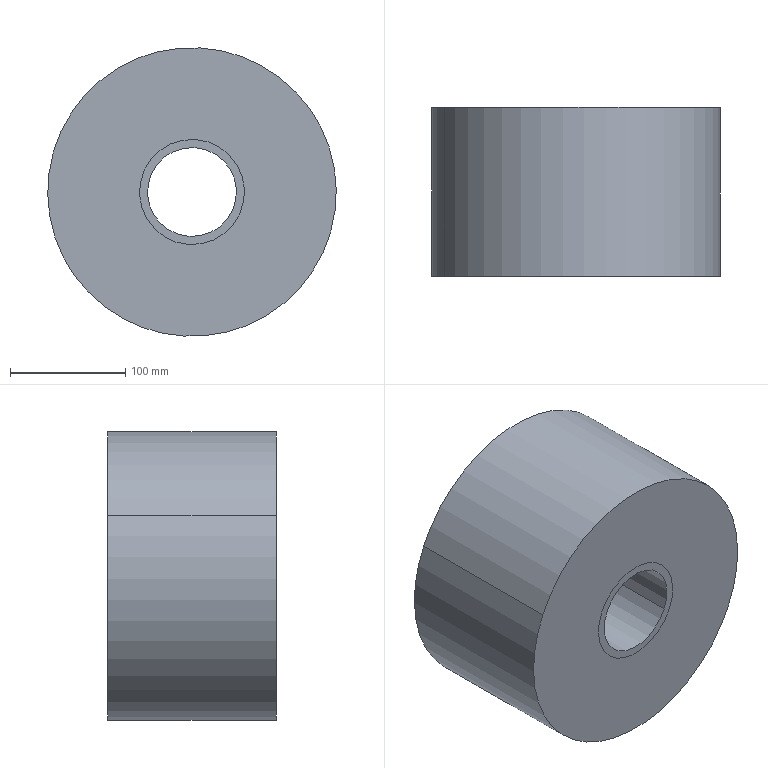Component | SolidWorks | ProtectiveFilm-4 | 2 solids | 12 faces | box 250 x 146 x 250 mm | volume 6486891 mm3 | cylinder 8 | plane 4 | commonest cylinder face diameters 91 x4 250 x2 77 x2
build123d program:
from build123d import *

# Parameters (mm, degrees)
SKETCH1_R           = 45.5
SKETCH1_R_2         = 38.5
BOSS_EXTRUDE1_DEPTH = 146
SKETCH2_R           = 125
SKETCH2_R_2         = 45.5
BOSS_EXTRUDE2_DEPTH = 146


with BuildPart() as part:
    # Sketch1 → Boss-Extrude1 (new body)
    with BuildSketch(Plane.XY):
        Circle(SKETCH1_R)
        Circle(SKETCH1_R_2, mode=Mode.SUBTRACT)
    extrude(amount=BOSS_EXTRUDE1_DEPTH)


with BuildPart() as body_2:
    # Sketch2 → Boss-Extrude2 (new body)
    with BuildSketch(Plane.XY):
        Circle(SKETCH2_R)
        Circle(SKETCH2_R_2, mode=Mode.SUBTRACT)
    extrude(amount=BOSS_EXTRUDE2_DEPTH)


solid = Compound([part.part, body_2.part])

# Placed as in the assembly
solid = solid.moved(Location((50, 183.5, 340), (90, 0, 0)))
STEP:
#1=COLOUR_RGB('',0.7922,0.8196,0.9333);
#2=FILL_AREA_STYLE_COLOUR('',#1);
#3=FILL_AREA_STYLE('',(#2));
#4=SURFACE_STYLE_FILL_AREA(#3);
#5=SURFACE_SIDE_STYLE('',(#4));
#6=SURFACE_STYLE_USAGE(.BOTH.,#5);
#7=PRESENTATION_STYLE_ASSIGNMENT((#6));
#8=CARTESIAN_POINT('',(0.3406,7.224,14.133));
#9=VERTEX_POINT('',#8);
#10=CARTESIAN_POINT('',(3.596,7.224,12.638));
#11=VERTEX_POINT('',#10);
#12=CARTESIAN_POINT('',(1.969,7.224,13.386));
#13=DIRECTION('',(0.,1.,0.));
#14=DIRECTION('',(0.9087,0.,-0.4174));
#15=AXIS2_PLACEMENT_3D('',#12,#13,#14);
#16=CIRCLE('',#15,1.791);
#17=EDGE_CURVE('',#9,#11,#16,.T.);
#18=ORIENTED_EDGE('',*,*,#17,.T.);
#19=CARTESIAN_POINT('',(3.596,1.476,12.638));
#20=VERTEX_POINT('',#19);
#21=CARTESIAN_POINT('',(3.596,7.224,12.638));
#22=DIRECTION('',(0.,-1.,0.));
#23=VECTOR('',#22,39.37);
#24=LINE('',#21,#23);
#25=EDGE_CURVE('',#11,#20,#24,.T.);
#26=ORIENTED_EDGE('',*,*,#25,.T.);
#27=CARTESIAN_POINT('',(0.3406,1.476,14.133));
#28=VERTEX_POINT('',#27);
#29=CARTESIAN_POINT('',(1.969,1.476,13.386));
#30=DIRECTION('',(0.,1.,0.));
#31=DIRECTION('',(0.9087,0.,-0.4174));
#32=AXIS2_PLACEMENT_3D('',#29,#30,#31);
#33=CIRCLE('',#32,1.791);
#34=EDGE_CURVE('',#28,#20,#33,.T.);
#35=ORIENTED_EDGE('',*,*,#34,.F.);
#36=CARTESIAN_POINT('',(0.3406,7.224,14.133));
#37=DIRECTION('',(0.,-1.,0.));
#38=VECTOR('',#37,39.37);
#39=LINE('',#36,#38);
#40=EDGE_CURVE('',#9,#28,#39,.T.);
#41=ORIENTED_EDGE('',*,*,#40,.F.);
#42=EDGE_LOOP('',(#18,#26,#35,#41));
#43=FACE_OUTER_BOUND('',#42,.T.);
#44=CARTESIAN_POINT('',(1.969,7.224,13.386));
#45=DIRECTION('',(0.,-1.,0.));
#46=DIRECTION('',(-0.9087,0.,0.4174));
#47=AXIS2_PLACEMENT_3D('',#44,#45,#46);
#48=CYLINDRICAL_SURFACE('',#47,1.791);
#49=ADVANCED_FACE('',(#43),#48,.F.);
#50=CARTESIAN_POINT('',(6.441,7.224,11.332));
#51=VERTEX_POINT('',#50);
#52=CARTESIAN_POINT('',(-2.504,7.224,15.44));
#53=VERTEX_POINT('',#52);
#54=CARTESIAN_POINT('',(1.969,7.224,13.386));
#55=DIRECTION('',(0.,1.,0.));
#56=DIRECTION('',(0.9087,0.,-0.4174));
#57=AXIS2_PLACEMENT_3D('',#54,#55,#56);
#58=CIRCLE('',#57,4.921);
#59=EDGE_CURVE('',#51,#53,#58,.T.);
#60=ORIENTED_EDGE('',*,*,#59,.F.);
#61=CARTESIAN_POINT('',(6.441,1.476,11.332));
#62=VERTEX_POINT('',#61);
#63=CARTESIAN_POINT('',(6.441,7.224,11.332));
#64=DIRECTION('',(0.,-1.,0.));
#65=VECTOR('',#64,39.37);
#66=LINE('',#63,#65);
#67=EDGE_CURVE('',#51,#62,#66,.T.);
#68=ORIENTED_EDGE('',*,*,#67,.T.);
#69=CARTESIAN_POINT('',(-2.504,1.476,15.44));
#70=VERTEX_POINT('',#69);
#71=CARTESIAN_POINT('',(1.969,1.476,13.386));
#72=DIRECTION('',(0.,1.,0.));
#73=DIRECTION('',(0.9087,0.,-0.4174));
#74=AXIS2_PLACEMENT_3D('',#71,#72,#73);
#75=CIRCLE('',#74,4.921);
#76=EDGE_CURVE('',#62,#70,#75,.T.);
#77=ORIENTED_EDGE('',*,*,#76,.T.);
#78=CARTESIAN_POINT('',(-2.504,7.224,15.44));
#79=DIRECTION('',(0.,-1.,0.));
#80=VECTOR('',#79,39.37);
#81=LINE('',#78,#80);
#82=EDGE_CURVE('',#53,#70,#81,.T.);
#83=ORIENTED_EDGE('',*,*,#82,.F.);
#84=EDGE_LOOP('',(#60,#68,#77,#83));
#85=FACE_OUTER_BOUND('',#84,.T.);
#86=CARTESIAN_POINT('',(1.969,7.224,13.386));
#87=DIRECTION('',(0.,-1.,0.));
#88=DIRECTION('',(-0.9087,0.,0.4174));
#89=AXIS2_PLACEMENT_3D('',#86,#87,#88);
#90=CYLINDRICAL_SURFACE('',#89,4.921);
#91=ADVANCED_FACE('',(#85),#90,.T.);
#92=CARTESIAN_POINT('',(1.969,7.224,13.386));
#93=DIRECTION('',(0.,1.,0.));
#94=DIRECTION('',(0.9087,0.,-0.4174));
#95=AXIS2_PLACEMENT_3D('',#92,#93,#94);
#96=CIRCLE('',#95,4.921);
#97=EDGE_CURVE('',#53,#51,#96,.T.);
#98=ORIENTED_EDGE('',*,*,#97,.T.);
#99=ORIENTED_EDGE('',*,*,#59,.T.);
#100=EDGE_LOOP('',(#98,#99));
#101=FACE_OUTER_BOUND('',#100,.T.);
#102=ORIENTED_EDGE('',*,*,#17,.F.);
#103=CARTESIAN_POINT('',(1.969,7.224,13.386));
#104=DIRECTION('',(0.,1.,0.));
#105=DIRECTION('',(0.9087,0.,-0.4174));
#106=AXIS2_PLACEMENT_3D('',#103,#104,#105);
#107=CIRCLE('',#106,1.791);
#108=EDGE_CURVE('',#11,#9,#107,.T.);
#109=ORIENTED_EDGE('',*,*,#108,.F.);
#110=EDGE_LOOP('',(#102,#109));
#111=FACE_BOUND('',#110,.T.);
#112=CARTESIAN_POINT('',(1.969,7.224,13.386));
#113=DIRECTION('',(0.,1.,0.));
#114=DIRECTION('',(0.9087,0.,-0.4174));
#115=AXIS2_PLACEMENT_3D('',#112,#113,#114);
#116=PLANE('',#115);
#117=ADVANCED_FACE('',(#101,#111),#116,.T.);
#118=CARTESIAN_POINT('',(1.969,1.476,13.386));
#119=DIRECTION('',(0.,1.,0.));
#120=DIRECTION('',(0.9087,0.,-0.4174));
#121=AXIS2_PLACEMENT_3D('',#118,#119,#120);
#122=CIRCLE('',#121,4.921);
#123=EDGE_CURVE('',#70,#62,#122,.T.);
#124=ORIENTED_EDGE('',*,*,#123,.F.);
#125=ORIENTED_EDGE('',*,*,#76,.F.);
#126=EDGE_LOOP('',(#124,#125));
#127=FACE_OUTER_BOUND('',#126,.T.);
#128=ORIENTED_EDGE('',*,*,#34,.T.);
#129=CARTESIAN_POINT('',(1.969,1.476,13.386));
#130=DIRECTION('',(0.,1.,0.));
#131=DIRECTION('',(0.9087,0.,-0.4174));
#132=AXIS2_PLACEMENT_3D('',#129,#130,#131);
#133=CIRCLE('',#132,1.791);
#134=EDGE_CURVE('',#20,#28,#133,.T.);
#135=ORIENTED_EDGE('',*,*,#134,.T.);
#136=EDGE_LOOP('',(#128,#135));
#137=FACE_BOUND('',#136,.T.);
#138=CARTESIAN_POINT('',(1.969,1.476,13.386));
#139=DIRECTION('',(0.,1.,0.));
#140=DIRECTION('',(0.9087,0.,-0.4174));
#141=AXIS2_PLACEMENT_3D('',#138,#139,#140);
#142=PLANE('',#141);
#143=ADVANCED_FACE('',(#127,#137),#142,.F.);
#144=ORIENTED_EDGE('',*,*,#67,.F.);
#145=ORIENTED_EDGE('',*,*,#97,.F.);
#146=ORIENTED_EDGE('',*,*,#82,.T.);
#147=ORIENTED_EDGE('',*,*,#123,.T.);
#148=EDGE_LOOP('',(#144,#145,#146,#147));
#149=FACE_OUTER_BOUND('',#148,.T.);
#150=CARTESIAN_POINT('',(1.969,7.224,13.386));
#151=DIRECTION('',(0.,-1.,0.));
#152=DIRECTION('',(-0.9087,0.,0.4174));
#153=AXIS2_PLACEMENT_3D('',#150,#151,#152);
#154=CYLINDRICAL_SURFACE('',#153,4.921);
#155=ADVANCED_FACE('',(#149),#154,.T.);
#156=ORIENTED_EDGE('',*,*,#25,.F.);
#157=ORIENTED_EDGE('',*,*,#108,.T.);
#158=ORIENTED_EDGE('',*,*,#40,.T.);
#159=ORIENTED_EDGE('',*,*,#134,.F.);
#160=EDGE_LOOP('',(#156,#157,#158,#159));
#161=FACE_OUTER_BOUND('',#160,.T.);
#162=CARTESIAN_POINT('',(1.969,7.224,13.386));
#163=DIRECTION('',(0.,-1.,0.));
#164=DIRECTION('',(-0.9087,0.,0.4174));
#165=AXIS2_PLACEMENT_3D('',#162,#163,#164);
#166=CYLINDRICAL_SURFACE('',#165,1.791);
#167=ADVANCED_FACE('',(#161),#166,.F.);
#168=CLOSED_SHELL('',(#49,#91,#117,#143,#155,#167));
#169=MANIFOLD_SOLID_BREP('',#168);
#170=STYLED_ITEM('',(#7),#169);
#171=(LENGTH_UNIT()NAMED_UNIT(*)SI_UNIT($,.METRE.));
#172=LENGTH_MEASURE_WITH_UNIT(LENGTH_MEASURE(0.0254),#171);
#173=DIMENSIONAL_EXPONENTS(1.,0.,0.,0.,0.,0.,0.);
#174=(CONVERSION_BASED_UNIT('',#172)LENGTH_UNIT()NAMED_UNIT(#173));
#175=UNCERTAINTY_MEASURE_WITH_UNIT(LENGTH_MEASURE(0.00001),#174,'','');
#176=(NAMED_UNIT(*)PLANE_ANGLE_UNIT()SI_UNIT($,.RADIAN.));
#177=(NAMED_UNIT(*)SI_UNIT($,.STERADIAN.)SOLID_ANGLE_UNIT());
#178=(GEOMETRIC_REPRESENTATION_CONTEXT(3)GLOBAL_UNCERTAINTY_ASSIGNED_CONTEXT((#175))GLOBAL_UNIT_ASSIGNED_CONTEXT((#174,#176,#177))REPRESENTATION_CONTEXT('',''));
#179=MECHANICAL_DESIGN_GEOMETRIC_PRESENTATION_REPRESENTATION('',(#170),#178);
#180=PRESENTATION_LAYER_ASSIGNMENT('','',(#170));
#181=CARTESIAN_POINT('',(0.5911,7.224,14.018));
#182=VERTEX_POINT('',#181);
#183=CARTESIAN_POINT('',(3.346,7.224,12.753));
#184=VERTEX_POINT('',#183);
#185=CARTESIAN_POINT('',(1.969,7.224,13.386));
#186=DIRECTION('',(0.,1.,0.));
#187=DIRECTION('',(0.9087,0.,-0.4174));
#188=AXIS2_PLACEMENT_3D('',#185,#186,#187);
#189=CIRCLE('',#188,1.516);
#190=EDGE_CURVE('',#182,#184,#189,.T.);
#191=ORIENTED_EDGE('',*,*,#190,.T.);
#192=CARTESIAN_POINT('',(3.346,1.476,12.753));
#193=VERTEX_POINT('',#192);
#194=CARTESIAN_POINT('',(3.346,7.224,12.753));
#195=DIRECTION('',(0.,-1.,0.));
#196=VECTOR('',#195,39.37);
#197=LINE('',#194,#196);
#198=EDGE_CURVE('',#184,#193,#197,.T.);
#199=ORIENTED_EDGE('',*,*,#198,.T.);
#200=CARTESIAN_POINT('',(0.5911,1.476,14.018));
#201=VERTEX_POINT('',#200);
#202=CARTESIAN_POINT('',(1.969,1.476,13.386));
#203=DIRECTION('',(0.,1.,0.));
#204=DIRECTION('',(0.9087,0.,-0.4174));
#205=AXIS2_PLACEMENT_3D('',#202,#203,#204);
#206=CIRCLE('',#205,1.516);
#207=EDGE_CURVE('',#201,#193,#206,.T.);
#208=ORIENTED_EDGE('',*,*,#207,.F.);
#209=CARTESIAN_POINT('',(0.5911,7.224,14.018));
#210=DIRECTION('',(0.,-1.,0.));
#211=VECTOR('',#210,39.37);
#212=LINE('',#209,#211);
#213=EDGE_CURVE('',#182,#201,#212,.T.);
#214=ORIENTED_EDGE('',*,*,#213,.F.);
#215=EDGE_LOOP('',(#191,#199,#208,#214));
#216=FACE_OUTER_BOUND('',#215,.T.);
#217=CARTESIAN_POINT('',(1.969,7.224,13.386));
#218=DIRECTION('',(0.,-1.,0.));
#219=DIRECTION('',(-0.9087,0.,0.4174));
#220=AXIS2_PLACEMENT_3D('',#217,#218,#219);
#221=CYLINDRICAL_SURFACE('',#220,1.516);
#222=ADVANCED_FACE('',(#216),#221,.F.);
#223=CARTESIAN_POINT('',(3.596,7.224,12.638));
#224=VERTEX_POINT('',#223);
#225=CARTESIAN_POINT('',(0.3406,7.224,14.133));
#226=VERTEX_POINT('',#225);
#227=CARTESIAN_POINT('',(1.969,7.224,13.386));
#228=DIRECTION('',(0.,1.,0.));
#229=DIRECTION('',(0.9087,0.,-0.4174));
#230=AXIS2_PLACEMENT_3D('',#227,#228,#229);
#231=CIRCLE('',#230,1.791);
#232=EDGE_CURVE('',#224,#226,#231,.T.);
#233=ORIENTED_EDGE('',*,*,#232,.F.);
#234=CARTESIAN_POINT('',(3.596,1.476,12.638));
#235=VERTEX_POINT('',#234);
#236=CARTESIAN_POINT('',(3.596,7.224,12.638));
#237=DIRECTION('',(0.,-1.,0.));
#238=VECTOR('',#237,39.37);
#239=LINE('',#236,#238);
#240=EDGE_CURVE('',#224,#235,#239,.T.);
#241=ORIENTED_EDGE('',*,*,#240,.T.);
#242=CARTESIAN_POINT('',(0.3406,1.476,14.133));
#243=VERTEX_POINT('',#242);
#244=CARTESIAN_POINT('',(1.969,1.476,13.386));
#245=DIRECTION('',(0.,1.,0.));
#246=DIRECTION('',(0.9087,0.,-0.4174));
#247=AXIS2_PLACEMENT_3D('',#244,#245,#246);
#248=CIRCLE('',#247,1.791);
#249=EDGE_CURVE('',#235,#243,#248,.T.);
#250=ORIENTED_EDGE('',*,*,#249,.T.);
#251=CARTESIAN_POINT('',(0.3406,7.224,14.133));
#252=DIRECTION('',(0.,-1.,0.));
#253=VECTOR('',#252,39.37);
#254=LINE('',#251,#253);
#255=EDGE_CURVE('',#226,#243,#254,.T.);
#256=ORIENTED_EDGE('',*,*,#255,.F.);
#257=EDGE_LOOP('',(#233,#241,#250,#256));
#258=FACE_OUTER_BOUND('',#257,.T.);
#259=CARTESIAN_POINT('',(1.969,7.224,13.386));
#260=DIRECTION('',(0.,-1.,0.));
#261=DIRECTION('',(-0.9087,0.,0.4174));
#262=AXIS2_PLACEMENT_3D('',#259,#260,#261);
#263=CYLINDRICAL_SURFACE('',#262,1.791);
#264=ADVANCED_FACE('',(#258),#263,.T.);
#265=CARTESIAN_POINT('',(1.969,7.224,13.386));
#266=DIRECTION('',(0.,1.,0.));
#267=DIRECTION('',(0.9087,0.,-0.4174));
#268=AXIS2_PLACEMENT_3D('',#265,#266,#267);
#269=CIRCLE('',#268,1.791);
#270=EDGE_CURVE('',#226,#224,#269,.T.);
#271=ORIENTED_EDGE('',*,*,#270,.T.);
#272=ORIENTED_EDGE('',*,*,#232,.T.);
#273=EDGE_LOOP('',(#271,#272));
#274=FACE_OUTER_BOUND('',#273,.T.);
#275=ORIENTED_EDGE('',*,*,#190,.F.);
#276=CARTESIAN_POINT('',(1.969,7.224,13.386));
#277=DIRECTION('',(0.,1.,0.));
#278=DIRECTION('',(0.9087,0.,-0.4174));
#279=AXIS2_PLACEMENT_3D('',#276,#277,#278);
#280=CIRCLE('',#279,1.516);
#281=EDGE_CURVE('',#184,#182,#280,.T.);
#282=ORIENTED_EDGE('',*,*,#281,.F.);
#283=EDGE_LOOP('',(#275,#282));
#284=FACE_BOUND('',#283,.T.);
#285=CARTESIAN_POINT('',(1.969,7.224,13.386));
#286=DIRECTION('',(0.,1.,0.));
#287=DIRECTION('',(0.9087,0.,-0.4174));
#288=AXIS2_PLACEMENT_3D('',#285,#286,#287);
#289=PLANE('',#288);
#290=ADVANCED_FACE('',(#274,#284),#289,.T.);
#291=CARTESIAN_POINT('',(1.969,1.476,13.386));
#292=DIRECTION('',(0.,1.,0.));
#293=DIRECTION('',(0.9087,0.,-0.4174));
#294=AXIS2_PLACEMENT_3D('',#291,#292,#293);
#295=CIRCLE('',#294,1.791);
#296=EDGE_CURVE('',#243,#235,#295,.T.);
#297=ORIENTED_EDGE('',*,*,#296,.F.);
#298=ORIENTED_EDGE('',*,*,#249,.F.);
#299=EDGE_LOOP('',(#297,#298));
#300=FACE_OUTER_BOUND('',#299,.T.);
#301=ORIENTED_EDGE('',*,*,#207,.T.);
#302=CARTESIAN_POINT('',(1.969,1.476,13.386));
#303=DIRECTION('',(0.,1.,0.));
#304=DIRECTION('',(0.9087,0.,-0.4174));
#305=AXIS2_PLACEMENT_3D('',#302,#303,#304);
#306=CIRCLE('',#305,1.516);
#307=EDGE_CURVE('',#193,#201,#306,.T.);
#308=ORIENTED_EDGE('',*,*,#307,.T.);
#309=EDGE_LOOP('',(#301,#308));
#310=FACE_BOUND('',#309,.T.);
#311=CARTESIAN_POINT('',(1.969,1.476,13.386));
#312=DIRECTION('',(0.,1.,0.));
#313=DIRECTION('',(0.9087,0.,-0.4174));
#314=AXIS2_PLACEMENT_3D('',#311,#312,#313);
#315=PLANE('',#314);
#316=ADVANCED_FACE('',(#300,#310),#315,.F.);
#317=ORIENTED_EDGE('',*,*,#240,.F.);
#318=ORIENTED_EDGE('',*,*,#270,.F.);
#319=ORIENTED_EDGE('',*,*,#255,.T.);
#320=ORIENTED_EDGE('',*,*,#296,.T.);
#321=EDGE_LOOP('',(#317,#318,#319,#320));
#322=FACE_OUTER_BOUND('',#321,.T.);
#323=CARTESIAN_POINT('',(1.969,7.224,13.386));
#324=DIRECTION('',(0.,-1.,0.));
#325=DIRECTION('',(-0.9087,0.,0.4174));
#326=AXIS2_PLACEMENT_3D('',#323,#324,#325);
#327=CYLINDRICAL_SURFACE('',#326,1.791);
#328=ADVANCED_FACE('',(#322),#327,.T.);
#329=ORIENTED_EDGE('',*,*,#198,.F.);
#330=ORIENTED_EDGE('',*,*,#281,.T.);
#331=ORIENTED_EDGE('',*,*,#213,.T.);
#332=ORIENTED_EDGE('',*,*,#307,.F.);
#333=EDGE_LOOP('',(#329,#330,#331,#332));
#334=FACE_OUTER_BOUND('',#333,.T.);
#335=CARTESIAN_POINT('',(1.969,7.224,13.386));
#336=DIRECTION('',(0.,-1.,0.));
#337=DIRECTION('',(-0.9087,0.,0.4174));
#338=AXIS2_PLACEMENT_3D('',#335,#336,#337);
#339=CYLINDRICAL_SURFACE('',#338,1.516);
#340=ADVANCED_FACE('',(#334),#339,.F.);
#341=CLOSED_SHELL('',(#222,#264,#290,#316,#328,#340));
#342=MANIFOLD_SOLID_BREP('',#341);
#343=CARTESIAN_POINT('',(0.,0.,0.));
#344=DIRECTION('',(0.,0.,1.));
#345=DIRECTION('',(1.,0.,0.));
#346=AXIS2_PLACEMENT_3D('',#343,#344,#345);
#347=(LENGTH_UNIT()NAMED_UNIT(*)SI_UNIT($,.METRE.));
#348=LENGTH_MEASURE_WITH_UNIT(LENGTH_MEASURE(0.0254),#347);
#349=DIMENSIONAL_EXPONENTS(1.,0.,0.,0.,0.,0.,0.);
#350=(CONVERSION_BASED_UNIT('',#348)LENGTH_UNIT()NAMED_UNIT(#349));
#351=UNCERTAINTY_MEASURE_WITH_UNIT(LENGTH_MEASURE(0.00001),#350,'','');
#352=(NAMED_UNIT(*)PLANE_ANGLE_UNIT()SI_UNIT($,.RADIAN.));
#353=(NAMED_UNIT(*)SI_UNIT($,.STERADIAN.)SOLID_ANGLE_UNIT());
#354=(GEOMETRIC_REPRESENTATION_CONTEXT(3)GLOBAL_UNCERTAINTY_ASSIGNED_CONTEXT((#351))GLOBAL_UNIT_ASSIGNED_CONTEXT((#350,#352,#353))REPRESENTATION_CONTEXT('',''));
#355=ADVANCED_BREP_SHAPE_REPRESENTATION('',(#169,#342,#346),#354);
#356=COLOUR_RGB('',0.7922,0.8196,0.9333);
#357=FILL_AREA_STYLE_COLOUR('',#356);
#358=FILL_AREA_STYLE('',(#357));
#359=SURFACE_STYLE_FILL_AREA(#358);
#360=SURFACE_SIDE_STYLE('',(#359));
#361=SURFACE_STYLE_USAGE(.BOTH.,#360);
#362=PRESENTATION_STYLE_ASSIGNMENT((#361));
#363=STYLED_ITEM('',(#362),#342);
#364=PRESENTATION_LAYER_ASSIGNMENT('','',(#363));
#365=(LENGTH_UNIT()NAMED_UNIT(*)SI_UNIT($,.METRE.));
#366=LENGTH_MEASURE_WITH_UNIT(LENGTH_MEASURE(0.0254),#365);
#367=DIMENSIONAL_EXPONENTS(1.,0.,0.,0.,0.,0.,0.);
#368=(CONVERSION_BASED_UNIT('',#366)LENGTH_UNIT()NAMED_UNIT(#367));
#369=UNCERTAINTY_MEASURE_WITH_UNIT(LENGTH_MEASURE(0.00001),#368,'','');
#370=(NAMED_UNIT(*)PLANE_ANGLE_UNIT()SI_UNIT($,.RADIAN.));
#371=(NAMED_UNIT(*)SI_UNIT($,.STERADIAN.)SOLID_ANGLE_UNIT());
#372=(GEOMETRIC_REPRESENTATION_CONTEXT(3)GLOBAL_UNCERTAINTY_ASSIGNED_CONTEXT((#369))GLOBAL_UNIT_ASSIGNED_CONTEXT((#368,#370,#371))REPRESENTATION_CONTEXT('',''));
#373=MECHANICAL_DESIGN_GEOMETRIC_PRESENTATION_REPRESENTATION('',(#363),#372);